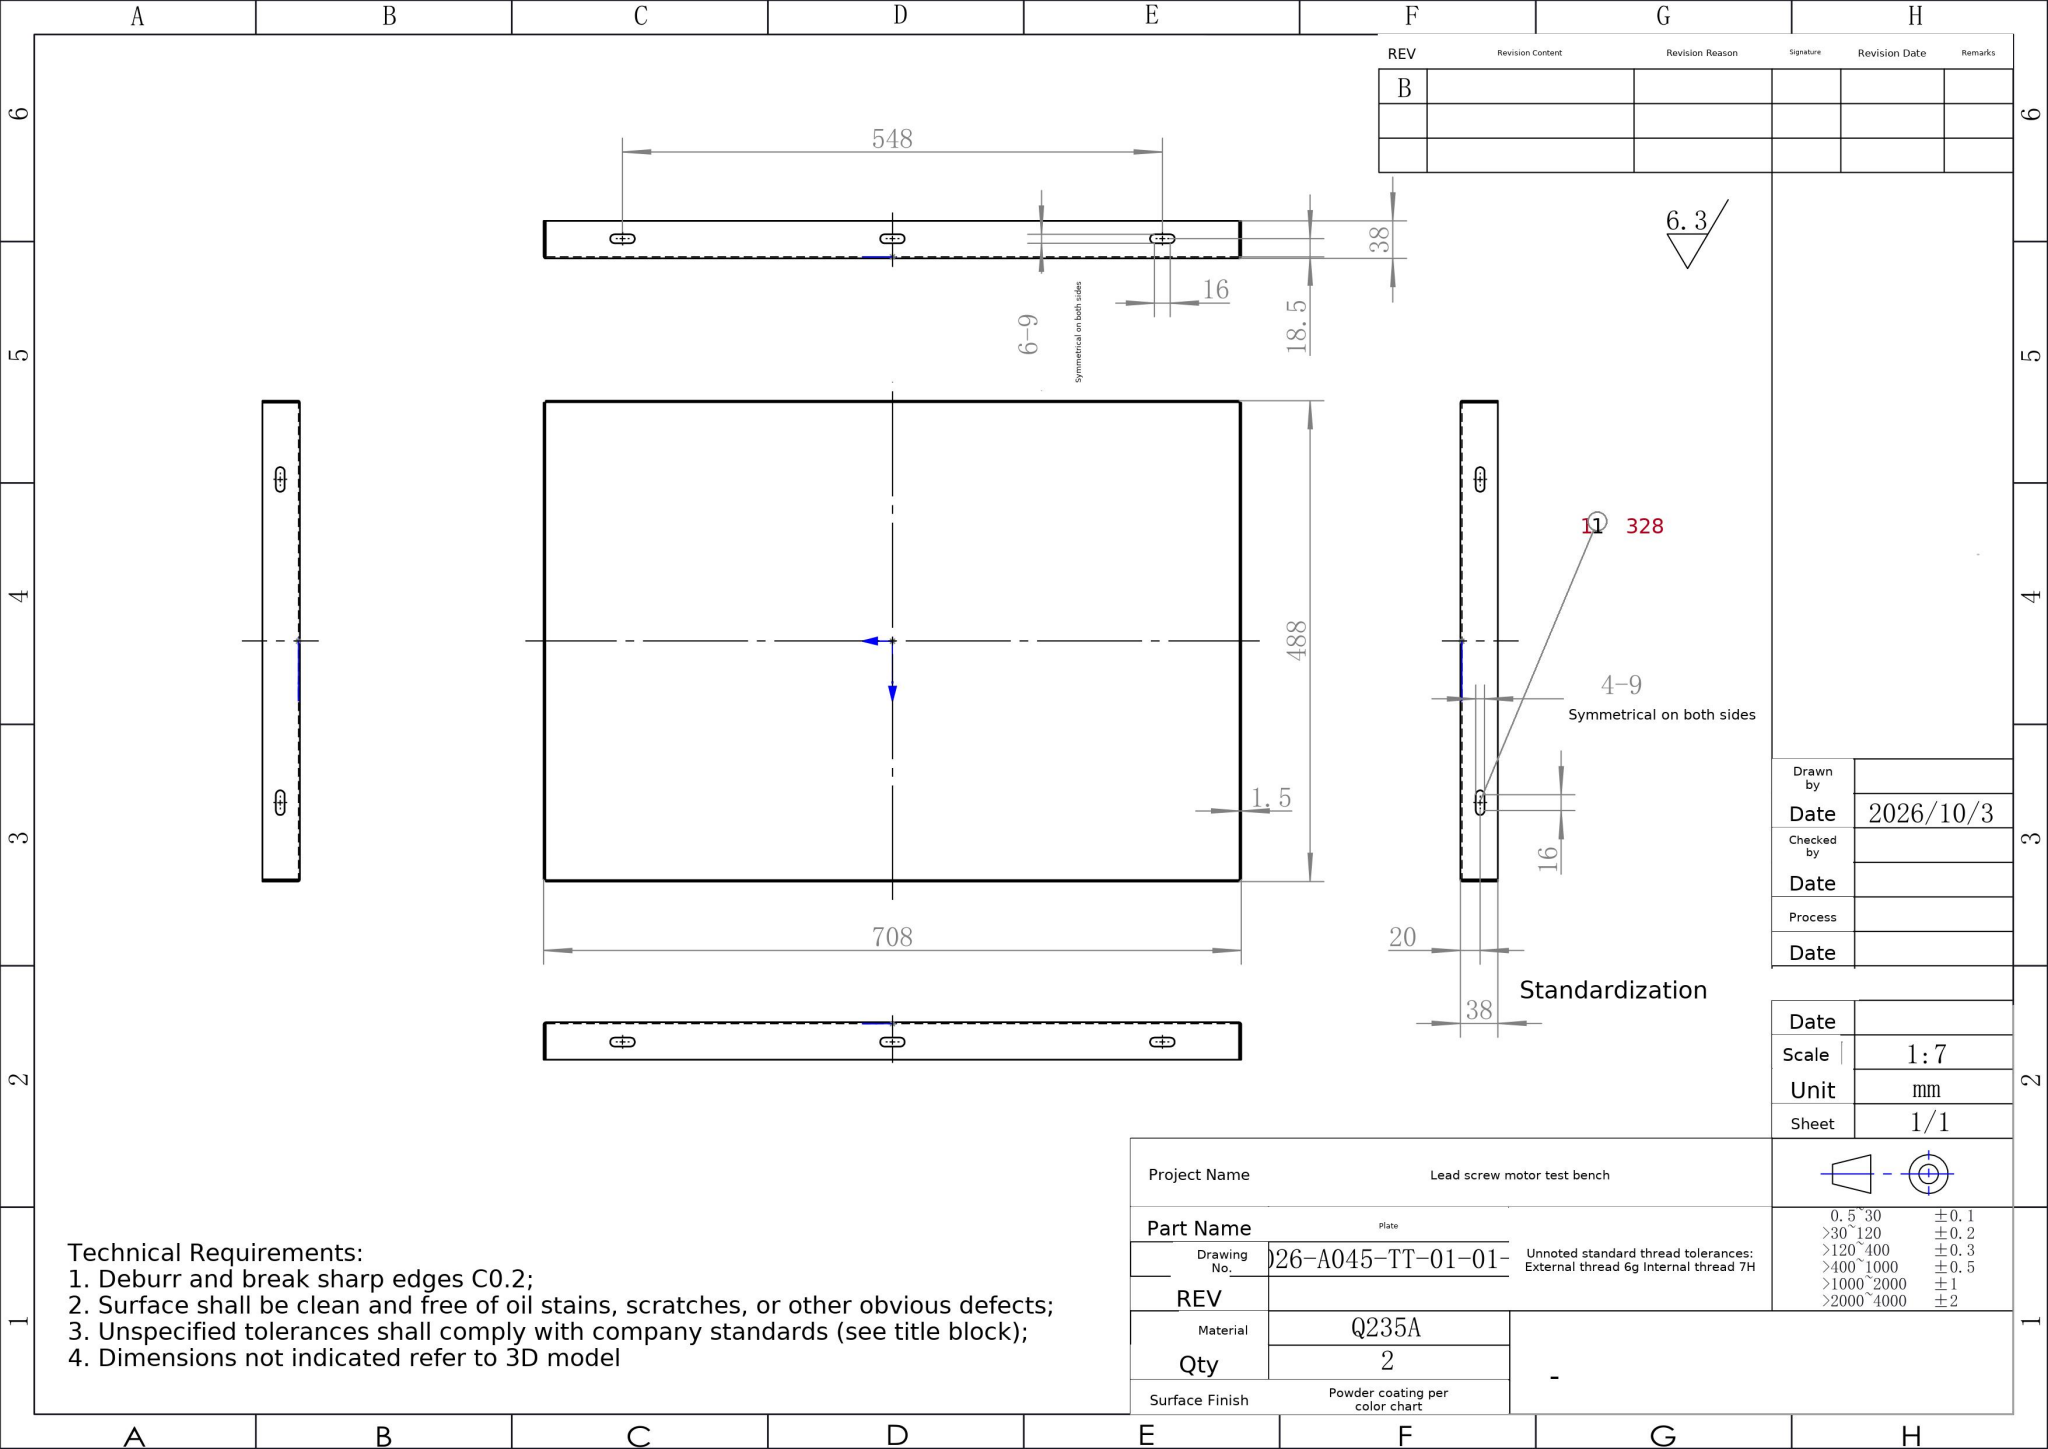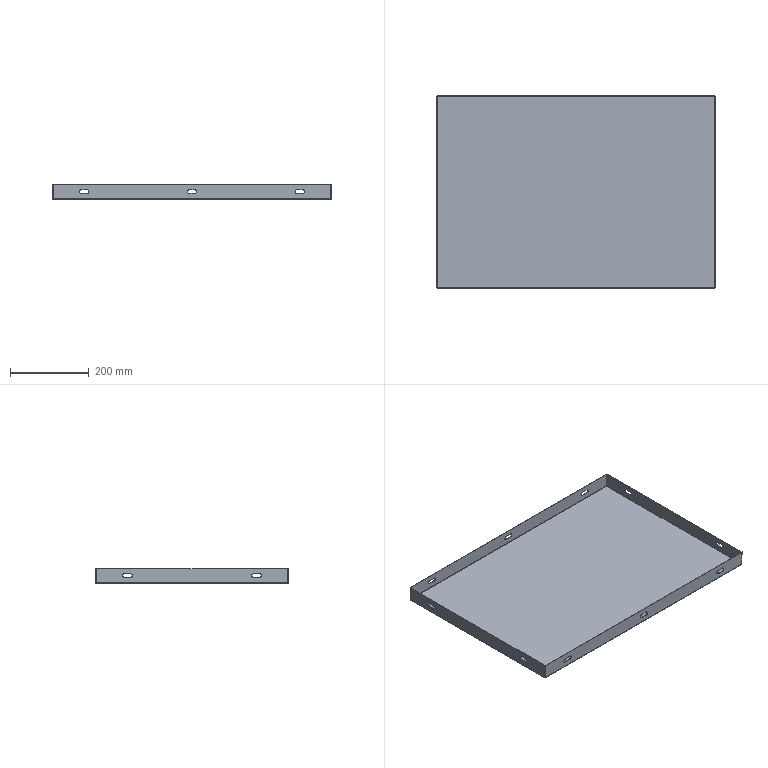Part | SolidWorks | mm | material Q235A | 1 solid | 78 faces | box 708 x 488 x 38 mm | volume 643200 mm3 | plane 42 | cylinder 28 | spline 8 | commonest cylinder face diameters 9 x20 4 x4 1 x4